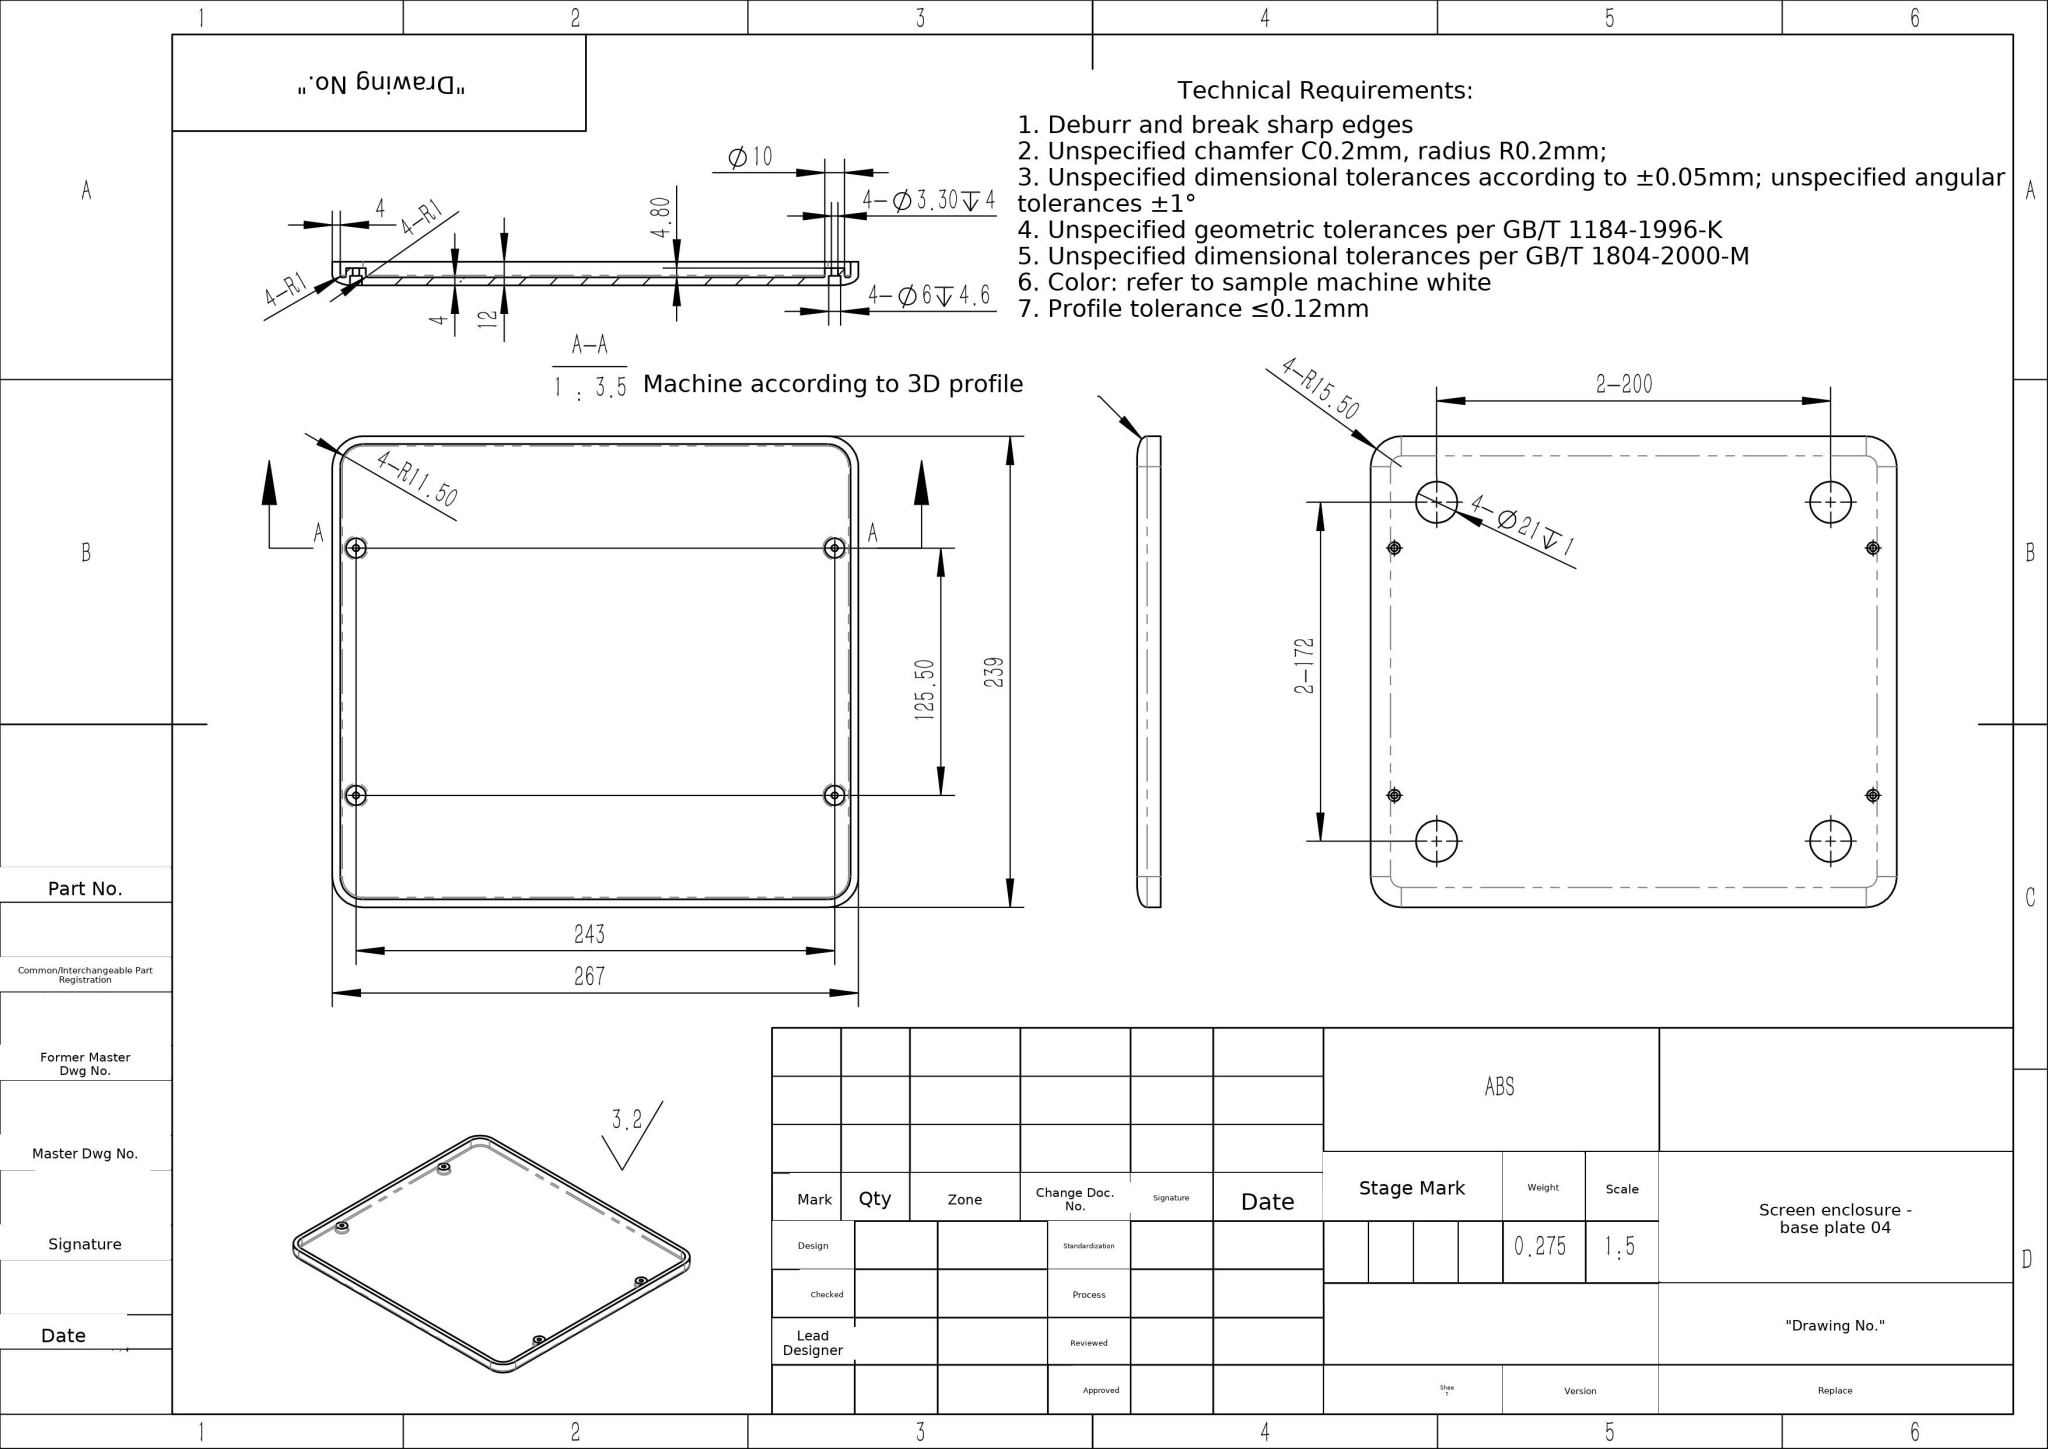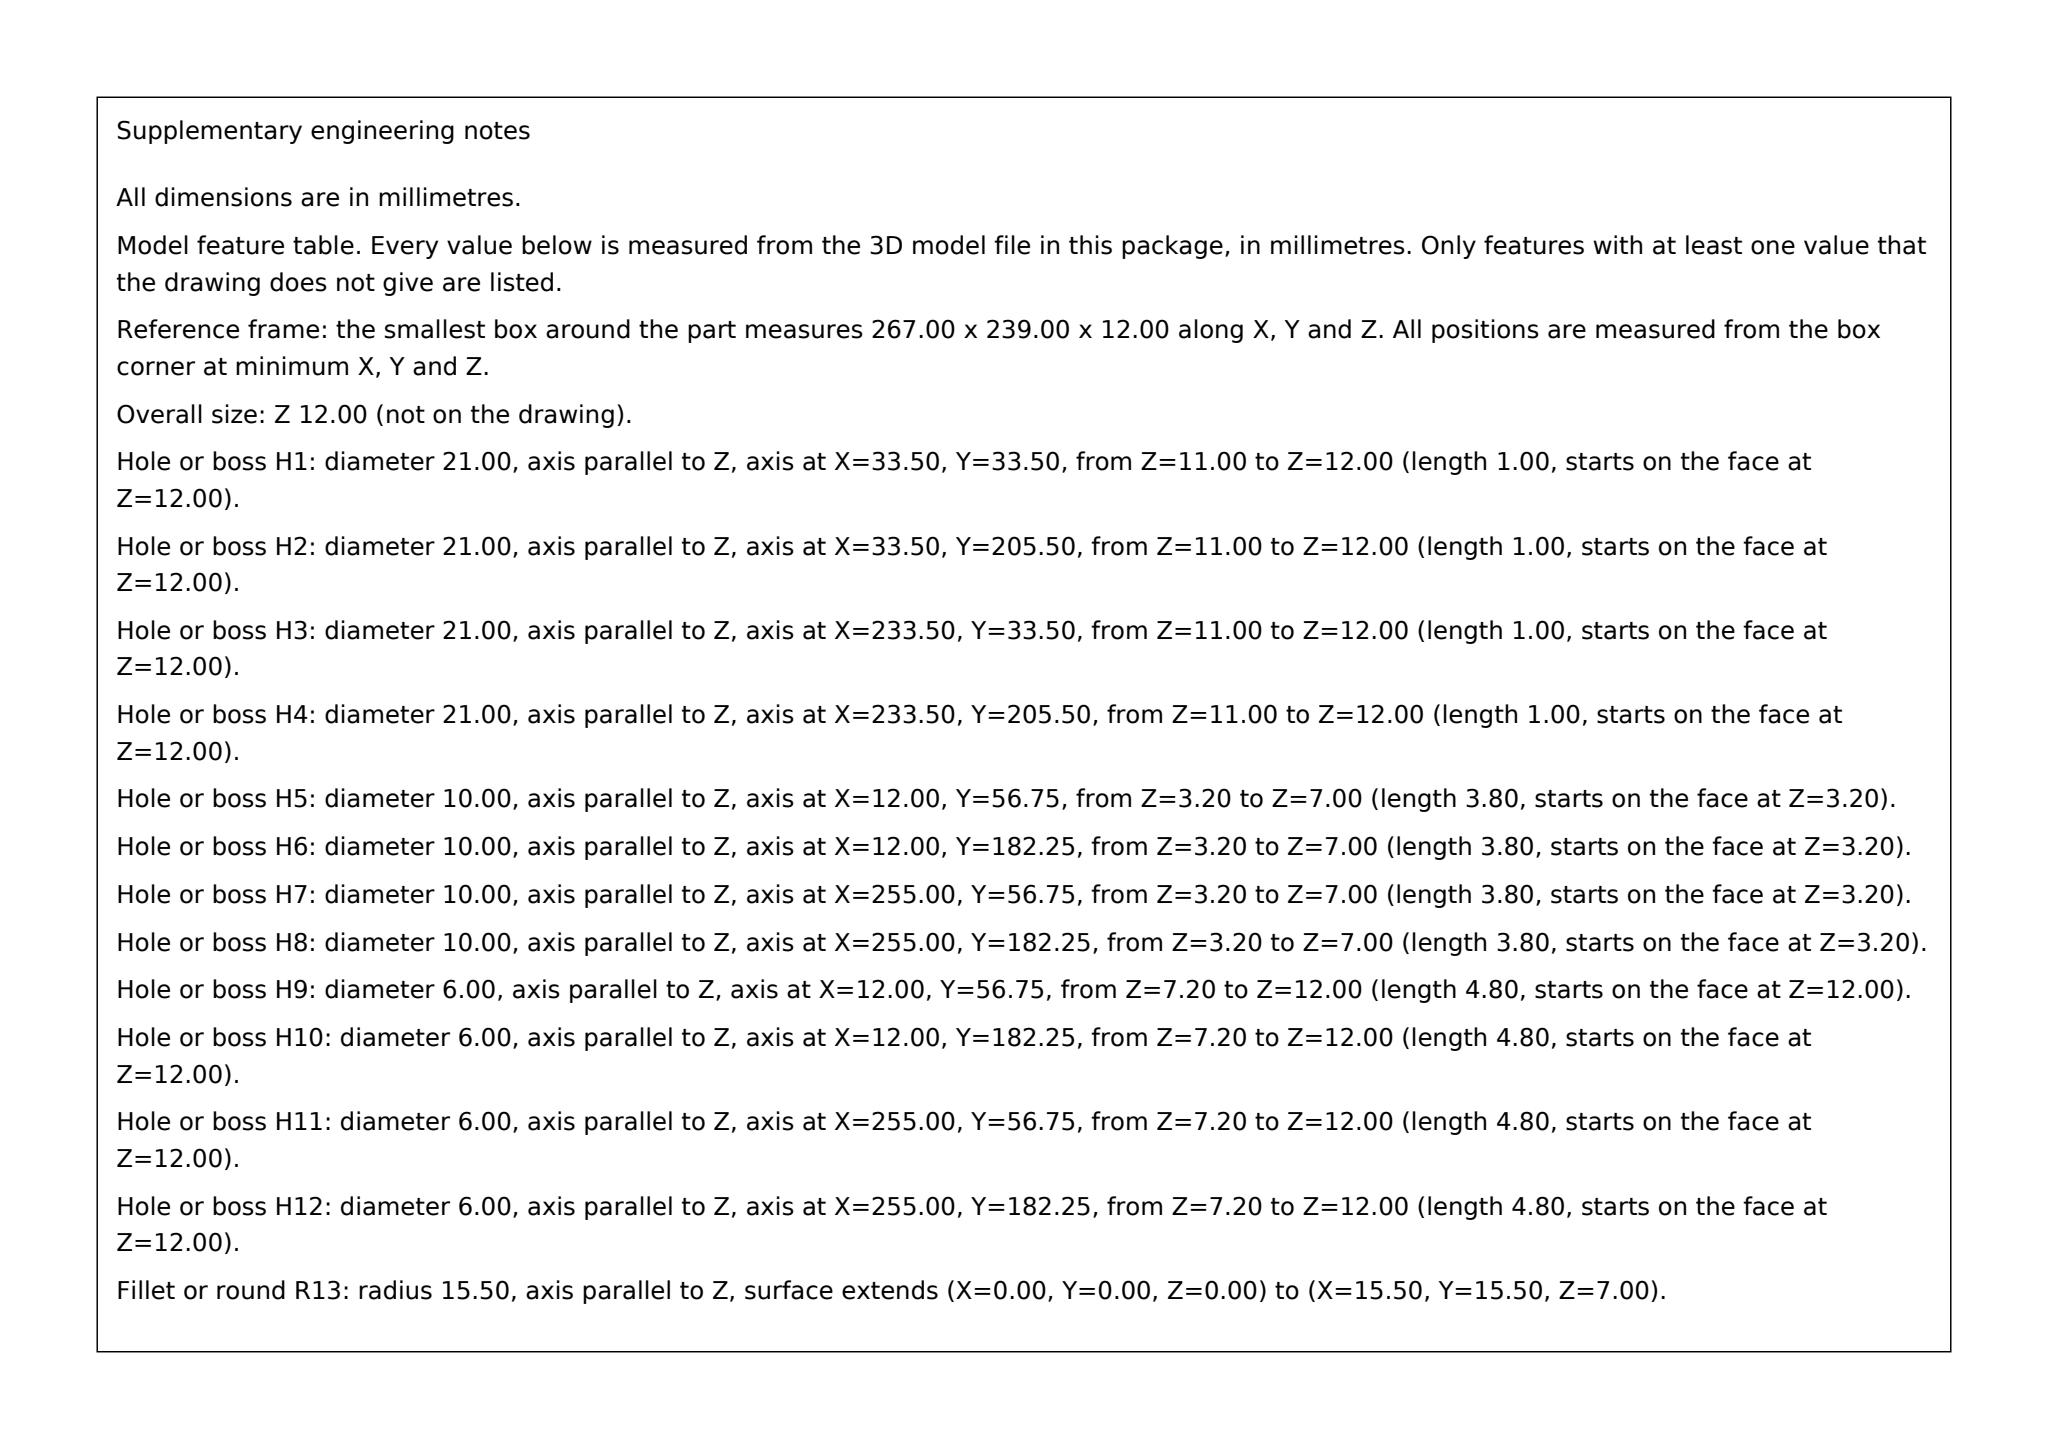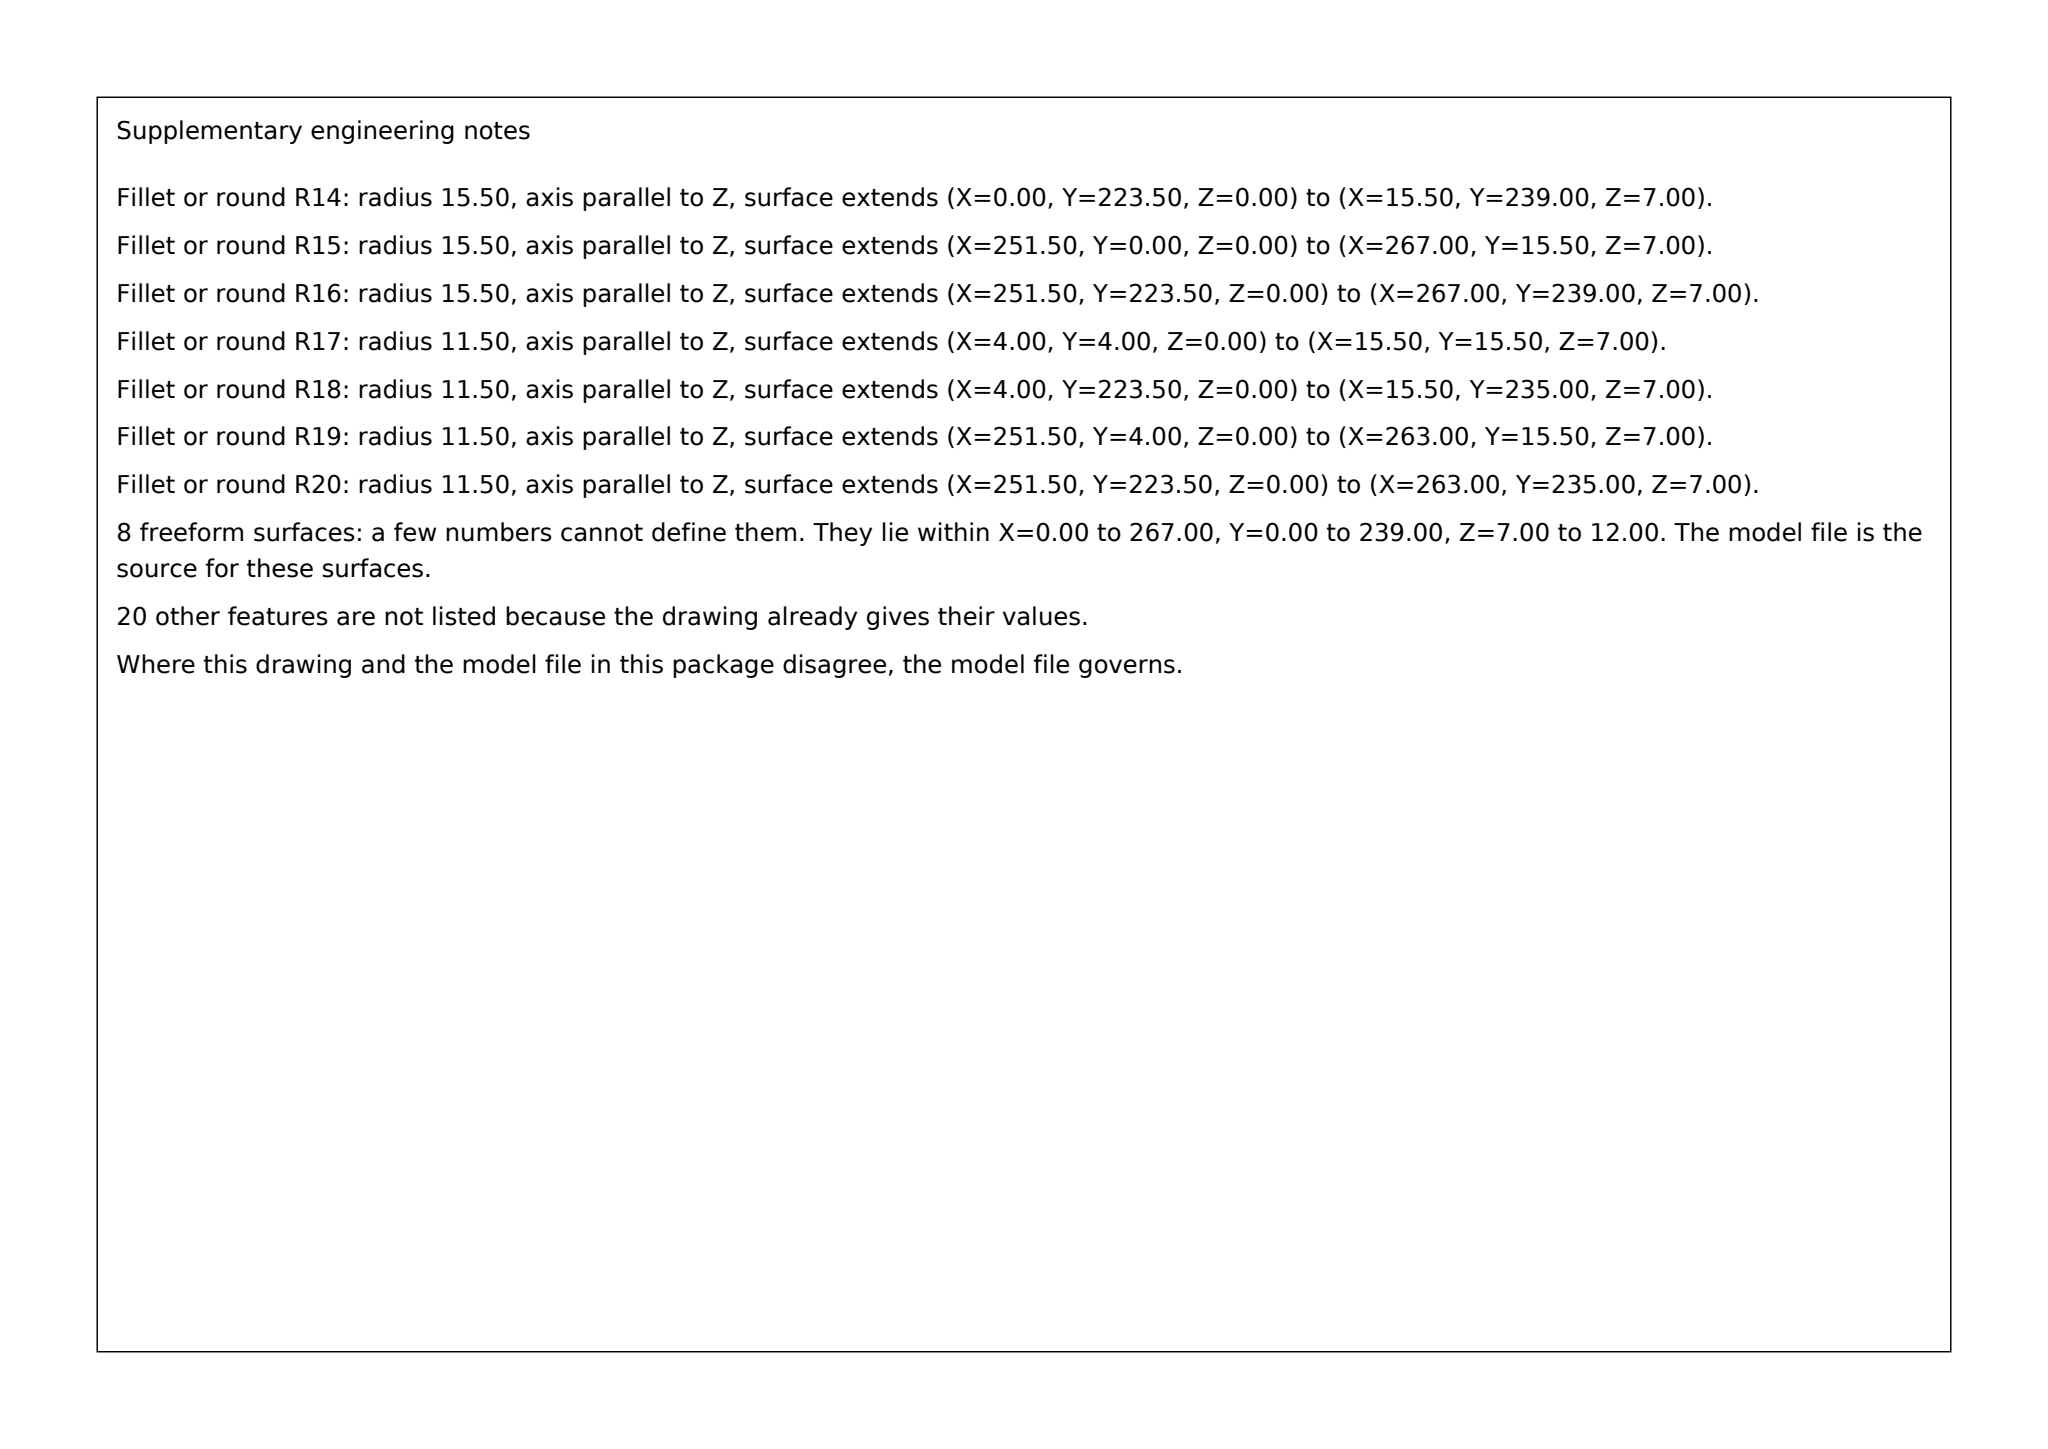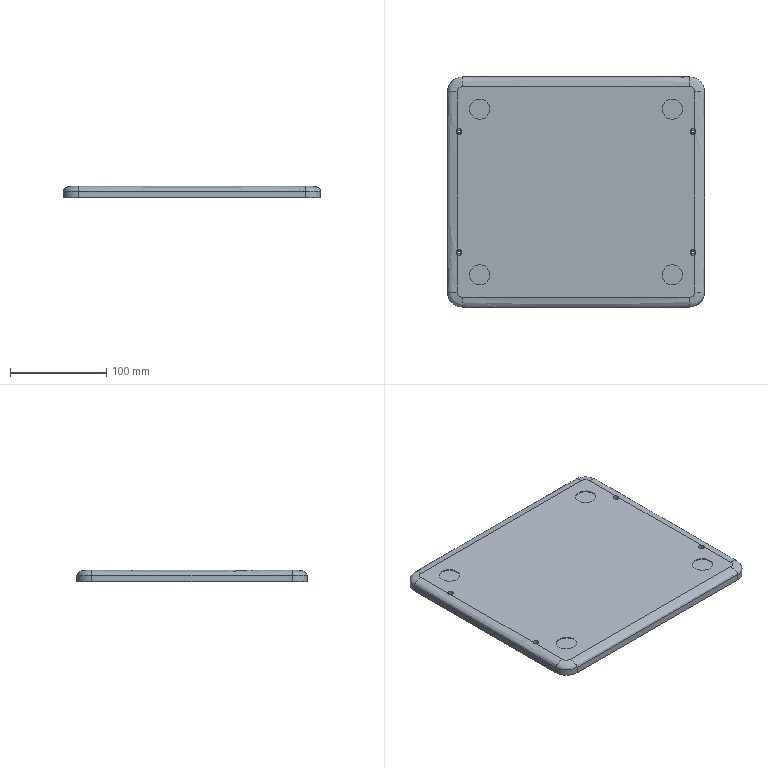Part | SolidWorks | mm | material ABS | 1 solid | 87 faces | box 267 x 239 x 12 mm | volume 274811 mm3 | cylinder 44 | plane 23 | torus 12 | spline 8 | commonest cylinder face diameters 6 x8 10 x8 21 x8 3.3 x8 31 x4 23 x4 2 x4